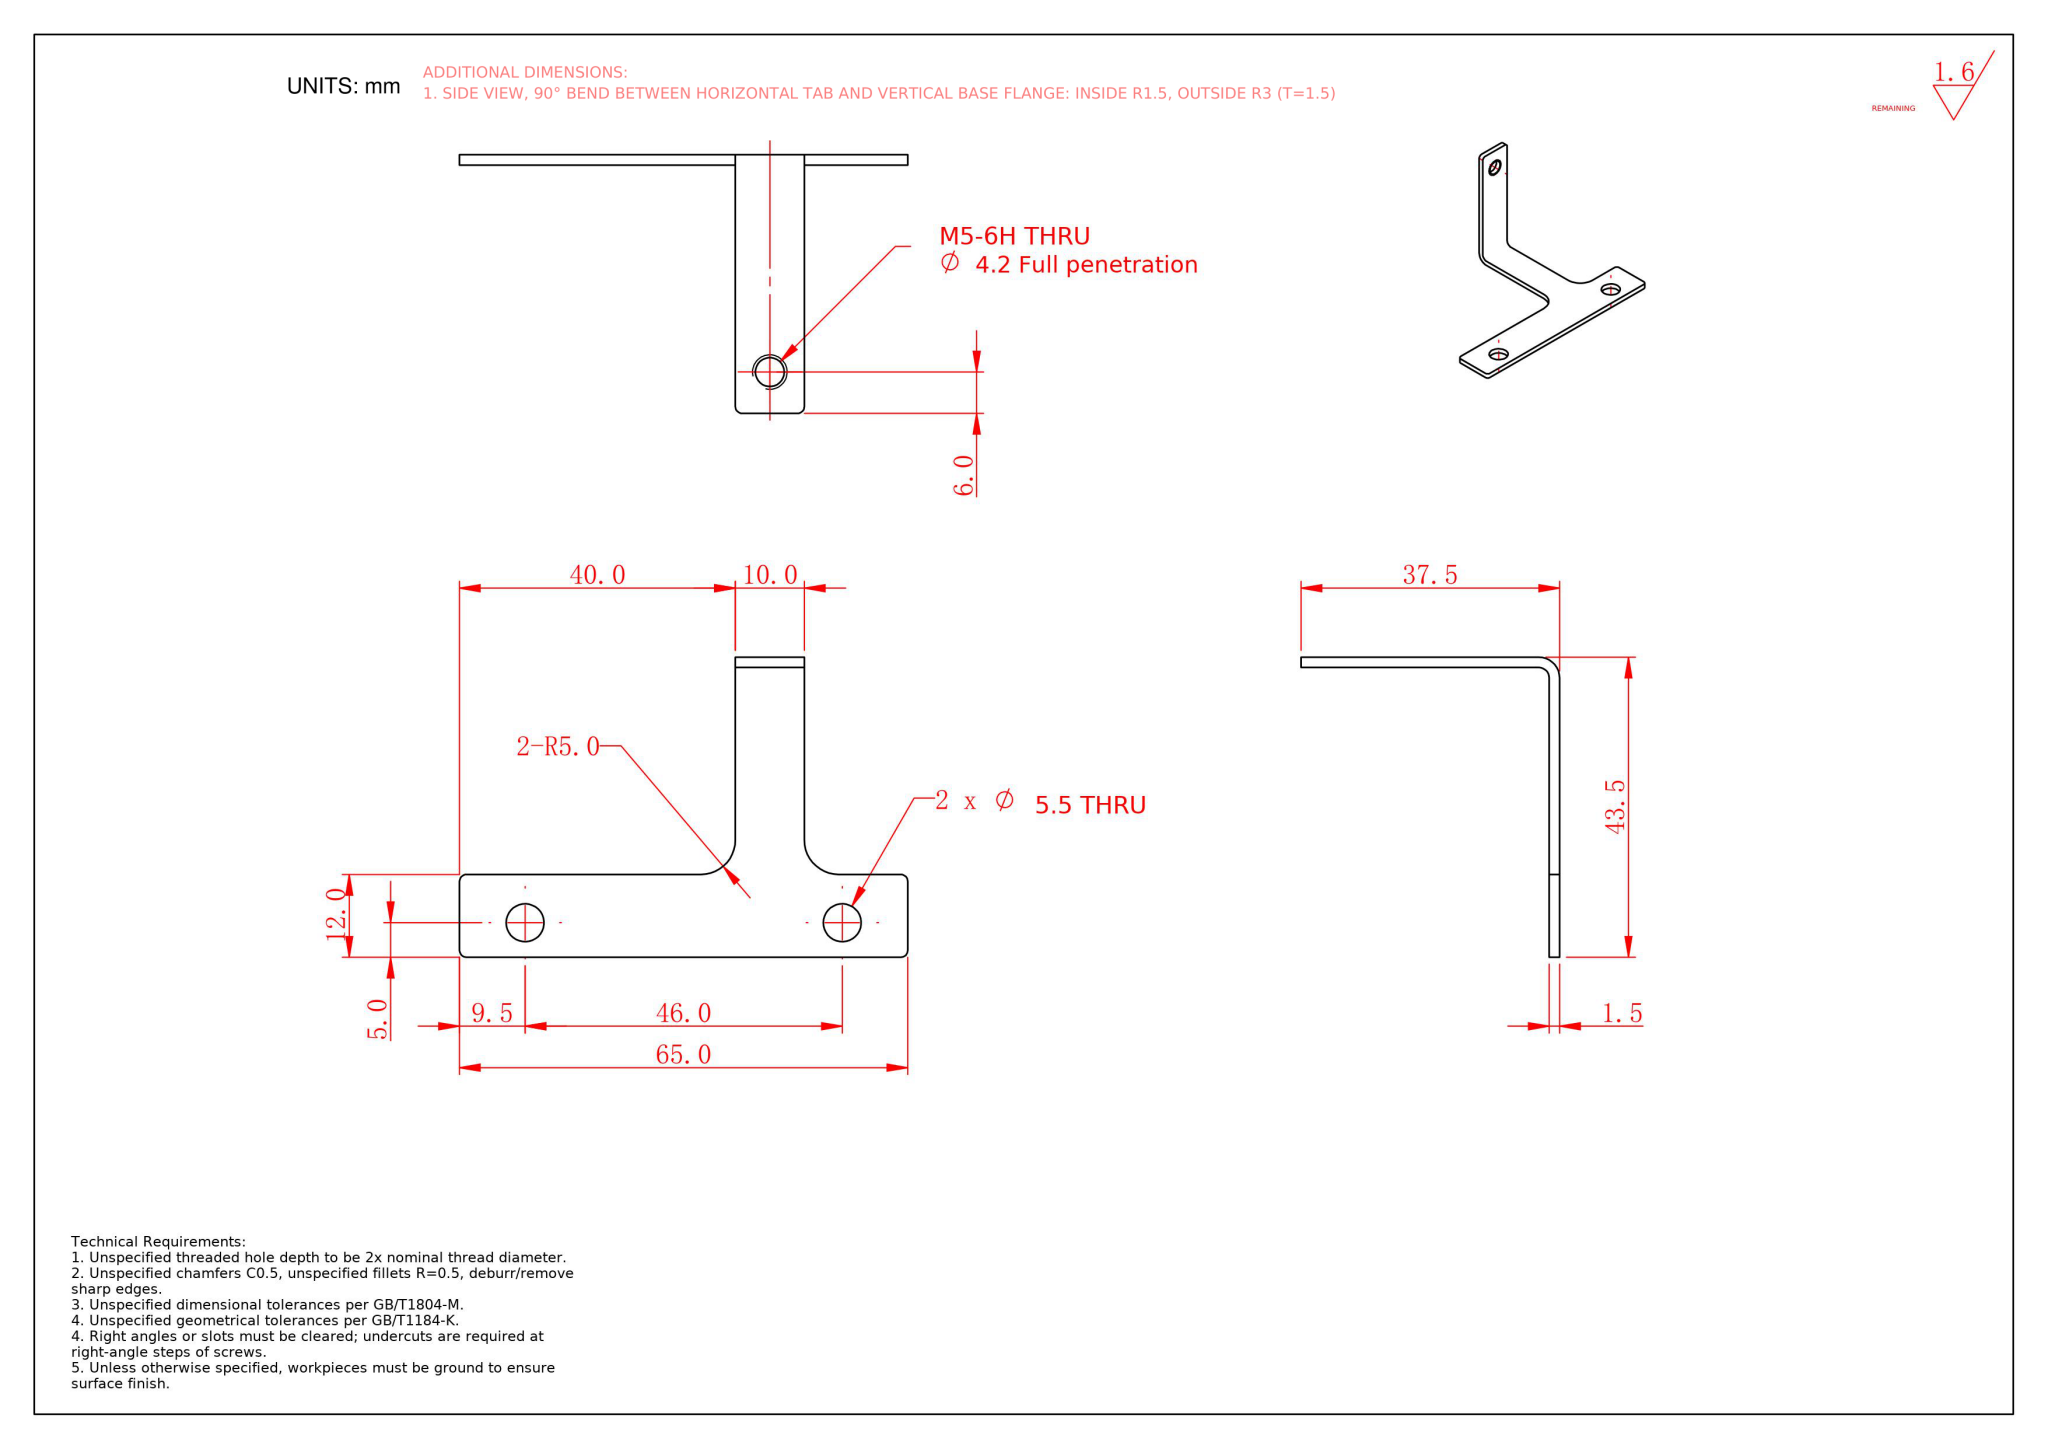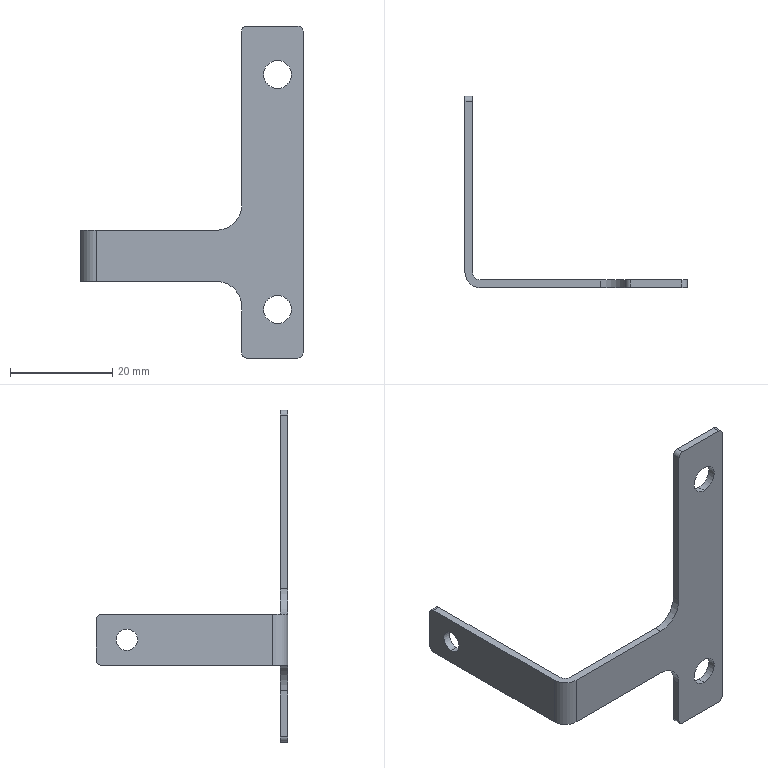Part | NX | mm | 1 solid | 28 faces | box 43.5 x 37.5 x 65 mm | volume 2090 mm3 | cylinder 16 | plane 12 | commonest cylinder face diameters 2 x6 5.5 x4 4.2 x2 10 x2 3 x1 6 x1
STEP:
#1=COLOUR_RGB('',1.,1.,1.);
#2=FILL_AREA_STYLE_COLOUR('',#1);
#3=FILL_AREA_STYLE('',(#2));
#4=SURFACE_STYLE_FILL_AREA(#3);
#5=SURFACE_SIDE_STYLE('',(#4));
#6=SURFACE_STYLE_USAGE(.BOTH.,#5);
#7=PRESENTATION_STYLE_ASSIGNMENT((#6));
#8=CARTESIAN_POINT('',(-27.384,150.278,52.75));
#9=VERTEX_POINT('',#8);
#10=CARTESIAN_POINT('',(-27.384,150.278,58.25));
#11=VERTEX_POINT('',#10);
#12=CARTESIAN_POINT('',(-27.384,150.278,55.5));
#13=DIRECTION('',(0.,1.,0.));
#14=DIRECTION('',(0.,0.,1.));
#15=AXIS2_PLACEMENT_3D('',#12,#13,#14);
#16=CIRCLE('',#15,2.75);
#17=EDGE_CURVE('',#9,#11,#16,.T.);
#18=ORIENTED_EDGE('',*,*,#17,.F.);
#19=CARTESIAN_POINT('',(-27.384,151.778,52.75));
#20=VERTEX_POINT('',#19);
#21=CARTESIAN_POINT('',(-27.384,151.778,52.75));
#22=DIRECTION('',(0.,1.,0.));
#23=VECTOR('',#22,1000.);
#24=LINE('',#21,#23);
#25=EDGE_CURVE('',#9,#20,#24,.T.);
#26=ORIENTED_EDGE('',*,*,#25,.T.);
#27=CARTESIAN_POINT('',(-27.384,151.778,58.25));
#28=VERTEX_POINT('',#27);
#29=CARTESIAN_POINT('',(-27.384,151.778,55.5));
#30=DIRECTION('',(0.,1.,0.));
#31=DIRECTION('',(0.,0.,1.));
#32=AXIS2_PLACEMENT_3D('',#29,#30,#31);
#33=CIRCLE('',#32,2.75);
#34=EDGE_CURVE('',#20,#28,#33,.T.);
#35=ORIENTED_EDGE('',*,*,#34,.T.);
#36=CARTESIAN_POINT('',(-27.384,151.778,58.25));
#37=DIRECTION('',(0.,1.,0.));
#38=VECTOR('',#37,1000.);
#39=LINE('',#36,#38);
#40=EDGE_CURVE('',#11,#28,#39,.T.);
#41=ORIENTED_EDGE('',*,*,#40,.F.);
#42=EDGE_LOOP('',(#18,#26,#35,#41));
#43=FACE_OUTER_BOUND('',#42,.T.);
#44=CARTESIAN_POINT('',(-27.384,151.778,55.5));
#45=DIRECTION('',(0.,1.,0.));
#46=DIRECTION('',(0.,0.,1.));
#47=AXIS2_PLACEMENT_3D('',#44,#45,#46);
#48=CYLINDRICAL_SURFACE('',#47,2.75);
#49=ADVANCED_FACE('',(#43),#48,.F.);
#50=CARTESIAN_POINT('',(-27.384,150.278,6.75));
#51=VERTEX_POINT('',#50);
#52=CARTESIAN_POINT('',(-27.384,150.278,12.25));
#53=VERTEX_POINT('',#52);
#54=CARTESIAN_POINT('',(-27.384,150.278,9.5));
#55=DIRECTION('',(0.,1.,0.));
#56=DIRECTION('',(0.,0.,1.));
#57=AXIS2_PLACEMENT_3D('',#54,#55,#56);
#58=CIRCLE('',#57,2.75);
#59=EDGE_CURVE('',#51,#53,#58,.T.);
#60=ORIENTED_EDGE('',*,*,#59,.F.);
#61=CARTESIAN_POINT('',(-27.384,151.778,6.75));
#62=VERTEX_POINT('',#61);
#63=CARTESIAN_POINT('',(-27.384,151.778,6.75));
#64=DIRECTION('',(0.,1.,0.));
#65=VECTOR('',#64,1000.);
#66=LINE('',#63,#65);
#67=EDGE_CURVE('',#51,#62,#66,.T.);
#68=ORIENTED_EDGE('',*,*,#67,.T.);
#69=CARTESIAN_POINT('',(-27.384,151.778,12.25));
#70=VERTEX_POINT('',#69);
#71=CARTESIAN_POINT('',(-27.384,151.778,9.5));
#72=DIRECTION('',(0.,1.,0.));
#73=DIRECTION('',(0.,0.,1.));
#74=AXIS2_PLACEMENT_3D('',#71,#72,#73);
#75=CIRCLE('',#74,2.75);
#76=EDGE_CURVE('',#62,#70,#75,.T.);
#77=ORIENTED_EDGE('',*,*,#76,.T.);
#78=CARTESIAN_POINT('',(-27.384,151.778,12.25));
#79=DIRECTION('',(0.,1.,0.));
#80=VECTOR('',#79,1000.);
#81=LINE('',#78,#80);
#82=EDGE_CURVE('',#53,#70,#81,.T.);
#83=ORIENTED_EDGE('',*,*,#82,.F.);
#84=EDGE_LOOP('',(#60,#68,#77,#83));
#85=FACE_OUTER_BOUND('',#84,.T.);
#86=CARTESIAN_POINT('',(-27.384,151.778,9.5));
#87=DIRECTION('',(0.,1.,0.));
#88=DIRECTION('',(0.,0.,1.));
#89=AXIS2_PLACEMENT_3D('',#86,#87,#88);
#90=CYLINDRICAL_SURFACE('',#89,2.75);
#91=ADVANCED_FACE('',(#85),#90,.F.);
#92=CARTESIAN_POINT('',(-65.884,181.778,22.1));
#93=VERTEX_POINT('',#92);
#94=CARTESIAN_POINT('',(-65.884,181.778,17.9));
#95=VERTEX_POINT('',#94);
#96=CARTESIAN_POINT('',(-65.884,181.778,20.));
#97=DIRECTION('',(1.,0.,0.));
#98=DIRECTION('',(0.,0.,-1.));
#99=AXIS2_PLACEMENT_3D('',#96,#97,#98);
#100=CIRCLE('',#99,2.1);
#101=EDGE_CURVE('',#93,#95,#100,.T.);
#102=ORIENTED_EDGE('',*,*,#101,.F.);
#103=CARTESIAN_POINT('',(-64.384,181.778,22.1));
#104=VERTEX_POINT('',#103);
#105=CARTESIAN_POINT('',(-64.384,181.778,22.1));
#106=DIRECTION('',(1.,0.,0.));
#107=VECTOR('',#106,1000.);
#108=LINE('',#105,#107);
#109=EDGE_CURVE('',#93,#104,#108,.T.);
#110=ORIENTED_EDGE('',*,*,#109,.T.);
#111=CARTESIAN_POINT('',(-64.384,181.778,17.9));
#112=VERTEX_POINT('',#111);
#113=CARTESIAN_POINT('',(-64.384,181.778,20.));
#114=DIRECTION('',(1.,0.,0.));
#115=DIRECTION('',(0.,0.,-1.));
#116=AXIS2_PLACEMENT_3D('',#113,#114,#115);
#117=CIRCLE('',#116,2.1);
#118=EDGE_CURVE('',#104,#112,#117,.T.);
#119=ORIENTED_EDGE('',*,*,#118,.T.);
#120=CARTESIAN_POINT('',(-64.384,181.778,17.9));
#121=DIRECTION('',(1.,0.,0.));
#122=VECTOR('',#121,1000.);
#123=LINE('',#120,#122);
#124=EDGE_CURVE('',#95,#112,#123,.T.);
#125=ORIENTED_EDGE('',*,*,#124,.F.);
#126=EDGE_LOOP('',(#102,#110,#119,#125));
#127=FACE_OUTER_BOUND('',#126,.T.);
#128=CARTESIAN_POINT('',(-64.384,181.778,20.));
#129=DIRECTION('',(1.,0.,0.));
#130=DIRECTION('',(0.,0.,-1.));
#131=AXIS2_PLACEMENT_3D('',#128,#129,#130);
#132=CYLINDRICAL_SURFACE('',#131,2.1);
#133=ADVANCED_FACE('',(#127),#132,.F.);
#134=CARTESIAN_POINT('',(-33.384,151.778,65.));
#135=VERTEX_POINT('',#134);
#136=CARTESIAN_POINT('',(-23.384,151.778,65.));
#137=VERTEX_POINT('',#136);
#138=CARTESIAN_POINT('',(-64.384,151.778,65.));
#139=DIRECTION('',(1.,0.,0.));
#140=VECTOR('',#139,1000.);
#141=LINE('',#138,#140);
#142=EDGE_CURVE('',#135,#137,#141,.T.);
#143=ORIENTED_EDGE('',*,*,#142,.F.);
#144=CARTESIAN_POINT('',(-33.384,150.278,65.));
#145=VERTEX_POINT('',#144);
#146=CARTESIAN_POINT('',(-33.384,150.278,65.));
#147=DIRECTION('',(0.,-1.,0.));
#148=VECTOR('',#147,1000.);
#149=LINE('',#146,#148);
#150=EDGE_CURVE('',#135,#145,#149,.T.);
#151=ORIENTED_EDGE('',*,*,#150,.T.);
#152=CARTESIAN_POINT('',(-23.384,150.278,65.));
#153=VERTEX_POINT('',#152);
#154=CARTESIAN_POINT('',(-64.384,150.278,65.));
#155=DIRECTION('',(1.,0.,0.));
#156=VECTOR('',#155,1000.);
#157=LINE('',#154,#156);
#158=EDGE_CURVE('',#145,#153,#157,.T.);
#159=ORIENTED_EDGE('',*,*,#158,.T.);
#160=CARTESIAN_POINT('',(-23.384,153.278,65.));
#161=DIRECTION('',(0.,1.,0.));
#162=VECTOR('',#161,1000.);
#163=LINE('',#160,#162);
#164=EDGE_CURVE('',#153,#137,#163,.T.);
#165=ORIENTED_EDGE('',*,*,#164,.T.);
#166=EDGE_LOOP('',(#143,#151,#159,#165));
#167=FACE_OUTER_BOUND('',#166,.T.);
#168=CARTESIAN_POINT('',(-65.884,153.278,65.));
#169=DIRECTION('',(0.,0.,1.));
#170=DIRECTION('',(1.,0.,0.));
#171=AXIS2_PLACEMENT_3D('',#168,#169,#170);
#172=PLANE('',#171);
#173=ADVANCED_FACE('',(#167),#172,.T.);
#174=CARTESIAN_POINT('',(-27.384,150.278,55.5));
#175=DIRECTION('',(0.,1.,0.));
#176=DIRECTION('',(0.,0.,1.));
#177=AXIS2_PLACEMENT_3D('',#174,#175,#176);
#178=CIRCLE('',#177,2.75);
#179=EDGE_CURVE('',#11,#9,#178,.T.);
#180=ORIENTED_EDGE('',*,*,#179,.T.);
#181=ORIENTED_EDGE('',*,*,#17,.T.);
#182=EDGE_LOOP('',(#180,#181));
#183=FACE_BOUND('',#182,.T.);
#184=CARTESIAN_POINT('',(-27.384,150.278,9.5));
#185=DIRECTION('',(0.,1.,0.));
#186=DIRECTION('',(0.,0.,1.));
#187=AXIS2_PLACEMENT_3D('',#184,#185,#186);
#188=CIRCLE('',#187,2.75);
#189=EDGE_CURVE('',#53,#51,#188,.T.);
#190=ORIENTED_EDGE('',*,*,#189,.T.);
#191=ORIENTED_EDGE('',*,*,#59,.T.);
#192=EDGE_LOOP('',(#190,#191));
#193=FACE_BOUND('',#192,.T.);
#194=CARTESIAN_POINT('',(-33.384,150.278,0.));
#195=VERTEX_POINT('',#194);
#196=CARTESIAN_POINT('',(-23.384,150.278,0.));
#197=VERTEX_POINT('',#196);
#198=CARTESIAN_POINT('',(-64.384,150.278,0.));
#199=DIRECTION('',(1.,0.,0.));
#200=VECTOR('',#199,1000.);
#201=LINE('',#198,#200);
#202=EDGE_CURVE('',#195,#197,#201,.T.);
#203=ORIENTED_EDGE('',*,*,#202,.T.);
#204=CARTESIAN_POINT('',(-22.384,150.278,1.));
#205=VERTEX_POINT('',#204);
#206=CARTESIAN_POINT('',(-23.384,150.278,1.));
#207=DIRECTION('',(0.,-1.,0.));
#208=DIRECTION('',(0.,0.,1.));
#209=AXIS2_PLACEMENT_3D('',#206,#207,#208);
#210=CIRCLE('',#209,1.);
#211=EDGE_CURVE('',#197,#205,#210,.T.);
#212=ORIENTED_EDGE('',*,*,#211,.T.);
#213=CARTESIAN_POINT('',(-22.384,150.278,64.));
#214=VERTEX_POINT('',#213);
#215=CARTESIAN_POINT('',(-22.384,150.278,65.));
#216=DIRECTION('',(0.,0.,-1.));
#217=VECTOR('',#216,1000.);
#218=LINE('',#215,#217);
#219=EDGE_CURVE('',#214,#205,#218,.T.);
#220=ORIENTED_EDGE('',*,*,#219,.F.);
#221=CARTESIAN_POINT('',(-23.384,150.278,64.));
#222=DIRECTION('',(0.,-1.,0.));
#223=DIRECTION('',(0.,0.,1.));
#224=AXIS2_PLACEMENT_3D('',#221,#222,#223);
#225=CIRCLE('',#224,1.);
#226=EDGE_CURVE('',#214,#153,#225,.T.);
#227=ORIENTED_EDGE('',*,*,#226,.T.);
#228=ORIENTED_EDGE('',*,*,#158,.F.);
#229=CARTESIAN_POINT('',(-34.384,150.278,64.));
#230=VERTEX_POINT('',#229);
#231=CARTESIAN_POINT('',(-33.384,150.278,64.));
#232=DIRECTION('',(0.,-1.,0.));
#233=DIRECTION('',(0.,0.,1.));
#234=AXIS2_PLACEMENT_3D('',#231,#232,#233);
#235=CIRCLE('',#234,1.);
#236=EDGE_CURVE('',#145,#230,#235,.T.);
#237=ORIENTED_EDGE('',*,*,#236,.T.);
#238=CARTESIAN_POINT('',(-34.384,150.278,30.));
#239=VERTEX_POINT('',#238);
#240=CARTESIAN_POINT('',(-34.384,150.278,79.419));
#241=DIRECTION('',(-0.,0.,-1.));
#242=VECTOR('',#241,1000.);
#243=LINE('',#240,#242);
#244=EDGE_CURVE('',#230,#239,#243,.T.);
#245=ORIENTED_EDGE('',*,*,#244,.T.);
#246=CARTESIAN_POINT('',(-39.384,150.278,25.));
#247=VERTEX_POINT('',#246);
#248=CARTESIAN_POINT('',(-39.384,150.278,30.));
#249=DIRECTION('',(0.,1.,0.));
#250=DIRECTION('',(0.,0.,1.));
#251=AXIS2_PLACEMENT_3D('',#248,#249,#250);
#252=CIRCLE('',#251,5.);
#253=EDGE_CURVE('',#239,#247,#252,.T.);
#254=ORIENTED_EDGE('',*,*,#253,.T.);
#255=CARTESIAN_POINT('',(-62.884,150.278,25.));
#256=VERTEX_POINT('',#255);
#257=CARTESIAN_POINT('',(-74.236,150.278,25.));
#258=DIRECTION('',(-1.,0.,0.));
#259=VECTOR('',#258,1000.);
#260=LINE('',#257,#259);
#261=EDGE_CURVE('',#247,#256,#260,.T.);
#262=ORIENTED_EDGE('',*,*,#261,.T.);
#263=CARTESIAN_POINT('',(-62.884,150.278,15.));
#264=VERTEX_POINT('',#263);
#265=CARTESIAN_POINT('',(-62.884,150.278,65.));
#266=DIRECTION('',(0.,0.,-1.));
#267=VECTOR('',#266,1000.);
#268=LINE('',#265,#267);
#269=EDGE_CURVE('',#256,#264,#268,.T.);
#270=ORIENTED_EDGE('',*,*,#269,.T.);
#271=CARTESIAN_POINT('',(-39.384,150.278,15.));
#272=VERTEX_POINT('',#271);
#273=CARTESIAN_POINT('',(-74.236,150.278,15.));
#274=DIRECTION('',(1.,0.,0.));
#275=VECTOR('',#274,1000.);
#276=LINE('',#273,#275);
#277=EDGE_CURVE('',#264,#272,#276,.T.);
#278=ORIENTED_EDGE('',*,*,#277,.T.);
#279=CARTESIAN_POINT('',(-34.384,150.278,10.));
#280=VERTEX_POINT('',#279);
#281=CARTESIAN_POINT('',(-39.384,150.278,10.));
#282=DIRECTION('',(0.,1.,0.));
#283=DIRECTION('',(0.,0.,1.));
#284=AXIS2_PLACEMENT_3D('',#281,#282,#283);
#285=CIRCLE('',#284,5.);
#286=EDGE_CURVE('',#272,#280,#285,.T.);
#287=ORIENTED_EDGE('',*,*,#286,.T.);
#288=CARTESIAN_POINT('',(-34.384,150.278,1.));
#289=VERTEX_POINT('',#288);
#290=CARTESIAN_POINT('',(-34.384,150.278,-20.192));
#291=DIRECTION('',(-0.,0.,-1.));
#292=VECTOR('',#291,1000.);
#293=LINE('',#290,#292);
#294=EDGE_CURVE('',#280,#289,#293,.T.);
#295=ORIENTED_EDGE('',*,*,#294,.T.);
#296=CARTESIAN_POINT('',(-33.384,150.278,1.));
#297=DIRECTION('',(0.,-1.,0.));
#298=DIRECTION('',(0.,0.,1.));
#299=AXIS2_PLACEMENT_3D('',#296,#297,#298);
#300=CIRCLE('',#299,1.);
#301=EDGE_CURVE('',#289,#195,#300,.T.);
#302=ORIENTED_EDGE('',*,*,#301,.T.);
#303=EDGE_LOOP('',(#203,#212,#220,#227,#228,#237,#245,#254,#262,#270,#278,#287,#295,#302));
#304=FACE_OUTER_BOUND('',#303,.T.);
#305=CARTESIAN_POINT('',(-64.384,150.278,65.));
#306=DIRECTION('',(0.,1.,0.));
#307=DIRECTION('',(0.,0.,1.));
#308=AXIS2_PLACEMENT_3D('',#305,#306,#307);
#309=PLANE('',#308);
#310=ADVANCED_FACE('',(#183,#193,#304),#309,.F.);
#311=ORIENTED_EDGE('',*,*,#219,.T.);
#312=CARTESIAN_POINT('',(-22.384,151.778,1.));
#313=VERTEX_POINT('',#312);
#314=CARTESIAN_POINT('',(-22.384,151.778,1.));
#315=DIRECTION('',(0.,1.,0.));
#316=VECTOR('',#315,1000.);
#317=LINE('',#314,#316);
#318=EDGE_CURVE('',#205,#313,#317,.T.);
#319=ORIENTED_EDGE('',*,*,#318,.T.);
#320=CARTESIAN_POINT('',(-22.384,151.778,64.));
#321=VERTEX_POINT('',#320);
#322=CARTESIAN_POINT('',(-22.384,151.778,65.));
#323=DIRECTION('',(0.,0.,-1.));
#324=VECTOR('',#323,1000.);
#325=LINE('',#322,#324);
#326=EDGE_CURVE('',#321,#313,#325,.T.);
#327=ORIENTED_EDGE('',*,*,#326,.F.);
#328=CARTESIAN_POINT('',(-22.384,151.778,64.));
#329=DIRECTION('',(0.,-1.,0.));
#330=VECTOR('',#329,1000.);
#331=LINE('',#328,#330);
#332=EDGE_CURVE('',#321,#214,#331,.T.);
#333=ORIENTED_EDGE('',*,*,#332,.T.);
#334=EDGE_LOOP('',(#311,#319,#327,#333));
#335=FACE_OUTER_BOUND('',#334,.T.);
#336=CARTESIAN_POINT('',(-22.384,151.778,65.));
#337=DIRECTION('',(1.,0.,0.));
#338=DIRECTION('',(0.,0.,-1.));
#339=AXIS2_PLACEMENT_3D('',#336,#337,#338);
#340=PLANE('',#339);
#341=ADVANCED_FACE('',(#335),#340,.T.);
#342=CARTESIAN_POINT('',(-27.384,151.778,55.5));
#343=DIRECTION('',(0.,1.,0.));
#344=DIRECTION('',(0.,0.,1.));
#345=AXIS2_PLACEMENT_3D('',#342,#343,#344);
#346=CIRCLE('',#345,2.75);
#347=EDGE_CURVE('',#28,#20,#346,.T.);
#348=ORIENTED_EDGE('',*,*,#347,.F.);
#349=ORIENTED_EDGE('',*,*,#34,.F.);
#350=EDGE_LOOP('',(#348,#349));
#351=FACE_BOUND('',#350,.T.);
#352=CARTESIAN_POINT('',(-27.384,151.778,9.5));
#353=DIRECTION('',(0.,1.,0.));
#354=DIRECTION('',(0.,0.,1.));
#355=AXIS2_PLACEMENT_3D('',#352,#353,#354);
#356=CIRCLE('',#355,2.75);
#357=EDGE_CURVE('',#70,#62,#356,.T.);
#358=ORIENTED_EDGE('',*,*,#357,.F.);
#359=ORIENTED_EDGE('',*,*,#76,.F.);
#360=EDGE_LOOP('',(#358,#359));
#361=FACE_BOUND('',#360,.T.);
#362=ORIENTED_EDGE('',*,*,#326,.T.);
#363=CARTESIAN_POINT('',(-23.384,151.778,0.));
#364=VERTEX_POINT('',#363);
#365=CARTESIAN_POINT('',(-23.384,151.778,1.));
#366=DIRECTION('',(0.,1.,0.));
#367=DIRECTION('',(0.,0.,1.));
#368=AXIS2_PLACEMENT_3D('',#365,#366,#367);
#369=CIRCLE('',#368,1.);
#370=EDGE_CURVE('',#313,#364,#369,.T.);
#371=ORIENTED_EDGE('',*,*,#370,.T.);
#372=CARTESIAN_POINT('',(-33.384,151.778,0.));
#373=VERTEX_POINT('',#372);
#374=CARTESIAN_POINT('',(-64.384,151.778,0.));
#375=DIRECTION('',(1.,0.,0.));
#376=VECTOR('',#375,1000.);
#377=LINE('',#374,#376);
#378=EDGE_CURVE('',#373,#364,#377,.T.);
#379=ORIENTED_EDGE('',*,*,#378,.F.);
#380=CARTESIAN_POINT('',(-34.384,151.778,1.));
#381=VERTEX_POINT('',#380);
#382=CARTESIAN_POINT('',(-33.384,151.778,1.));
#383=DIRECTION('',(0.,1.,0.));
#384=DIRECTION('',(0.,0.,1.));
#385=AXIS2_PLACEMENT_3D('',#382,#383,#384);
#386=CIRCLE('',#385,1.);
#387=EDGE_CURVE('',#373,#381,#386,.T.);
#388=ORIENTED_EDGE('',*,*,#387,.T.);
#389=CARTESIAN_POINT('',(-34.384,151.778,10.));
#390=VERTEX_POINT('',#389);
#391=CARTESIAN_POINT('',(-34.384,151.778,65.));
#392=DIRECTION('',(-0.,0.,-1.));
#393=VECTOR('',#392,1000.);
#394=LINE('',#391,#393);
#395=EDGE_CURVE('',#390,#381,#394,.T.);
#396=ORIENTED_EDGE('',*,*,#395,.F.);
#397=CARTESIAN_POINT('',(-39.384,151.778,15.));
#398=VERTEX_POINT('',#397);
#399=CARTESIAN_POINT('',(-39.384,151.778,10.));
#400=DIRECTION('',(0.,-1.,0.));
#401=DIRECTION('',(-0.,0.,1.));
#402=AXIS2_PLACEMENT_3D('',#399,#400,#401);
#403=CIRCLE('',#402,5.);
#404=EDGE_CURVE('',#390,#398,#403,.T.);
#405=ORIENTED_EDGE('',*,*,#404,.T.);
#406=CARTESIAN_POINT('',(-62.884,151.778,15.));
#407=VERTEX_POINT('',#406);
#408=CARTESIAN_POINT('',(-64.384,151.778,15.));
#409=DIRECTION('',(1.,0.,0.));
#410=VECTOR('',#409,1000.);
#411=LINE('',#408,#410);
#412=EDGE_CURVE('',#407,#398,#411,.T.);
#413=ORIENTED_EDGE('',*,*,#412,.F.);
#414=CARTESIAN_POINT('',(-62.884,151.778,25.));
#415=VERTEX_POINT('',#414);
#416=CARTESIAN_POINT('',(-62.884,151.778,65.));
#417=DIRECTION('',(0.,0.,-1.));
#418=VECTOR('',#417,1000.);
#419=LINE('',#416,#418);
#420=EDGE_CURVE('',#415,#407,#419,.T.);
#421=ORIENTED_EDGE('',*,*,#420,.F.);
#422=CARTESIAN_POINT('',(-39.384,151.778,25.));
#423=VERTEX_POINT('',#422);
#424=CARTESIAN_POINT('',(-64.384,151.778,25.));
#425=DIRECTION('',(-1.,0.,0.));
#426=VECTOR('',#425,1000.);
#427=LINE('',#424,#426);
#428=EDGE_CURVE('',#423,#415,#427,.T.);
#429=ORIENTED_EDGE('',*,*,#428,.F.);
#430=CARTESIAN_POINT('',(-34.384,151.778,30.));
#431=VERTEX_POINT('',#430);
#432=CARTESIAN_POINT('',(-39.384,151.778,30.));
#433=DIRECTION('',(0.,-1.,0.));
#434=DIRECTION('',(0.,0.,1.));
#435=AXIS2_PLACEMENT_3D('',#432,#433,#434);
#436=CIRCLE('',#435,5.);
#437=EDGE_CURVE('',#423,#431,#436,.T.);
#438=ORIENTED_EDGE('',*,*,#437,.T.);
#439=CARTESIAN_POINT('',(-34.384,151.778,64.));
#440=VERTEX_POINT('',#439);
#441=CARTESIAN_POINT('',(-34.384,151.778,65.));
#442=DIRECTION('',(-0.,0.,-1.));
#443=VECTOR('',#442,1000.);
#444=LINE('',#441,#443);
#445=EDGE_CURVE('',#440,#431,#444,.T.);
#446=ORIENTED_EDGE('',*,*,#445,.F.);
#447=CARTESIAN_POINT('',(-33.384,151.778,64.));
#448=DIRECTION('',(0.,1.,0.));
#449=DIRECTION('',(0.,0.,1.));
#450=AXIS2_PLACEMENT_3D('',#447,#448,#449);
#451=CIRCLE('',#450,1.);
#452=EDGE_CURVE('',#440,#135,#451,.T.);
#453=ORIENTED_EDGE('',*,*,#452,.T.);
#454=ORIENTED_EDGE('',*,*,#142,.T.);
#455=CARTESIAN_POINT('',(-23.384,151.778,64.));
#456=DIRECTION('',(0.,1.,0.));
#457=DIRECTION('',(0.,0.,1.));
#458=AXIS2_PLACEMENT_3D('',#455,#456,#457);
#459=CIRCLE('',#458,1.);
#460=EDGE_CURVE('',#137,#321,#459,.T.);
#461=ORIENTED_EDGE('',*,*,#460,.T.);
#462=EDGE_LOOP('',(#362,#371,#379,#388,#396,#405,#413,#421,#429,#438,#446,#453,#454,#461));
#463=FACE_OUTER_BOUND('',#462,.T.);
#464=CARTESIAN_POINT('',(-64.384,151.778,65.));
#465=DIRECTION('',(0.,1.,0.));
#466=DIRECTION('',(0.,0.,1.));
#467=AXIS2_PLACEMENT_3D('',#464,#465,#466);
#468=PLANE('',#467);
#469=ADVANCED_FACE('',(#351,#361,#463),#468,.T.);
#470=CARTESIAN_POINT('',(-64.384,153.278,25.));
#471=VERTEX_POINT('',#470);
#472=CARTESIAN_POINT('',(-62.884,153.278,25.));
#473=DIRECTION('',(0.,0.,-1.));
#474=DIRECTION('',(-1.,0.,0.));
#475=AXIS2_PLACEMENT_3D('',#472,#473,#474);
#476=CIRCLE('',#475,1.5);
#477=EDGE_CURVE('',#415,#471,#476,.T.);
#478=ORIENTED_EDGE('',*,*,#477,.F.);
#479=ORIENTED_EDGE('',*,*,#420,.T.);
#480=CARTESIAN_POINT('',(-64.384,153.278,15.));
#481=VERTEX_POINT('',#480);
#482=CARTESIAN_POINT('',(-62.884,153.278,15.));
#483=DIRECTION('',(0.,0.,1.));
#484=DIRECTION('',(1.,0.,0.));
#485=AXIS2_PLACEMENT_3D('',#482,#483,#484);
#486=CIRCLE('',#485,1.5);
#487=EDGE_CURVE('',#481,#407,#486,.T.);
#488=ORIENTED_EDGE('',*,*,#487,.F.);
#489=CARTESIAN_POINT('',(-64.384,153.278,65.));
#490=DIRECTION('',(0.,0.,-1.));
#491=VECTOR('',#490,1000.);
#492=LINE('',#489,#491);
#493=EDGE_CURVE('',#471,#481,#492,.T.);
#494=ORIENTED_EDGE('',*,*,#493,.F.);
#495=EDGE_LOOP('',(#478,#479,#488,#494));
#496=FACE_OUTER_BOUND('',#495,.T.);
#497=CARTESIAN_POINT('',(-62.884,153.278,65.));
#498=DIRECTION('',(0.,0.,-1.));
#499=DIRECTION('',(-1.,0.,0.));
#500=AXIS2_PLACEMENT_3D('',#497,#498,#499);
#501=CYLINDRICAL_SURFACE('',#500,1.5);
#502=ADVANCED_FACE('',(#496),#501,.F.);
#503=CARTESIAN_POINT('',(-64.384,181.778,20.));
#504=DIRECTION('',(1.,0.,0.));
#505=DIRECTION('',(0.,0.,-1.));
#506=AXIS2_PLACEMENT_3D('',#503,#504,#505);
#507=CIRCLE('',#506,2.1);
#508=EDGE_CURVE('',#112,#104,#507,.T.);
#509=ORIENTED_EDGE('',*,*,#508,.F.);
#510=ORIENTED_EDGE('',*,*,#118,.F.);
#511=EDGE_LOOP('',(#509,#510));
#512=FACE_BOUND('',#511,.T.);
#513=CARTESIAN_POINT('',(-64.384,186.778,15.));
#514=VERTEX_POINT('',#513);
#515=CARTESIAN_POINT('',(-64.384,187.778,15.));
#516=DIRECTION('',(0.,-1.,0.));
#517=VECTOR('',#516,1000.);
#518=LINE('',#515,#517);
#519=EDGE_CURVE('',#514,#481,#518,.T.);
#520=ORIENTED_EDGE('',*,*,#519,.F.);
#521=CARTESIAN_POINT('',(-64.384,187.778,16.));
#522=VERTEX_POINT('',#521);
#523=CARTESIAN_POINT('',(-64.384,186.778,16.));
#524=DIRECTION('',(1.,0.,0.));
#525=DIRECTION('',(0.,1.,0.));
#526=AXIS2_PLACEMENT_3D('',#523,#524,#525);
#527=CIRCLE('',#526,1.);
#528=EDGE_CURVE('',#514,#522,#527,.T.);
#529=ORIENTED_EDGE('',*,*,#528,.T.);
#530=CARTESIAN_POINT('',(-64.384,187.778,24.));
#531=VERTEX_POINT('',#530);
#532=CARTESIAN_POINT('',(-64.384,187.778,65.));
#533=DIRECTION('',(0.,0.,-1.));
#534=VECTOR('',#533,1000.);
#535=LINE('',#532,#534);
#536=EDGE_CURVE('',#531,#522,#535,.T.);
#537=ORIENTED_EDGE('',*,*,#536,.F.);
#538=CARTESIAN_POINT('',(-64.384,186.778,25.));
#539=VERTEX_POINT('',#538);
#540=CARTESIAN_POINT('',(-64.384,186.778,24.));
#541=DIRECTION('',(1.,0.,0.));
#542=DIRECTION('',(0.,1.,0.));
#543=AXIS2_PLACEMENT_3D('',#540,#541,#542);
#544=CIRCLE('',#543,1.);
#545=EDGE_CURVE('',#531,#539,#544,.T.);
#546=ORIENTED_EDGE('',*,*,#545,.T.);
#547=CARTESIAN_POINT('',(-64.384,187.778,25.));
#548=DIRECTION('',(-0.,1.,0.));
#549=VECTOR('',#548,1000.);
#550=LINE('',#547,#549);
#551=EDGE_CURVE('',#471,#539,#550,.T.);
#552=ORIENTED_EDGE('',*,*,#551,.F.);
#553=ORIENTED_EDGE('',*,*,#493,.T.);
#554=EDGE_LOOP('',(#520,#529,#537,#546,#552,#553));
#555=FACE_OUTER_BOUND('',#554,.T.);
#556=CARTESIAN_POINT('',(-64.384,187.778,65.));
#557=DIRECTION('',(1.,0.,0.));
#558=DIRECTION('',(-0.,1.,0.));
#559=AXIS2_PLACEMENT_3D('',#556,#557,#558);
#560=PLANE('',#559);
#561=ADVANCED_FACE('',(#512,#555),#560,.T.);
#562=ORIENTED_EDGE('',*,*,#536,.T.);
#563=CARTESIAN_POINT('',(-65.884,187.778,16.));
#564=VERTEX_POINT('',#563);
#565=CARTESIAN_POINT('',(-65.884,187.778,16.));
#566=DIRECTION('',(-1.,0.,0.));
#567=VECTOR('',#566,1000.);
#568=LINE('',#565,#567);
#569=EDGE_CURVE('',#522,#564,#568,.T.);
#570=ORIENTED_EDGE('',*,*,#569,.T.);
#571=CARTESIAN_POINT('',(-65.884,187.778,24.));
#572=VERTEX_POINT('',#571);
#573=CARTESIAN_POINT('',(-65.884,187.778,65.));
#574=DIRECTION('',(0.,0.,-1.));
#575=VECTOR('',#574,1000.);
#576=LINE('',#573,#575);
#577=EDGE_CURVE('',#572,#564,#576,.T.);
#578=ORIENTED_EDGE('',*,*,#577,.F.);
#579=CARTESIAN_POINT('',(-64.384,187.778,24.));
#580=DIRECTION('',(1.,0.,0.));
#581=VECTOR('',#580,1000.);
#582=LINE('',#579,#581);
#583=EDGE_CURVE('',#572,#531,#582,.T.);
#584=ORIENTED_EDGE('',*,*,#583,.T.);
#585=EDGE_LOOP('',(#562,#570,#578,#584));
#586=FACE_OUTER_BOUND('',#585,.T.);
#587=CARTESIAN_POINT('',(-65.884,187.778,65.));
#588=DIRECTION('',(0.,1.,0.));
#589=DIRECTION('',(0.,0.,1.));
#590=AXIS2_PLACEMENT_3D('',#587,#588,#589);
#591=PLANE('',#590);
#592=ADVANCED_FACE('',(#586),#591,.T.);
#593=CARTESIAN_POINT('',(-65.884,181.778,20.));
#594=DIRECTION('',(1.,0.,0.));
#595=DIRECTION('',(0.,0.,-1.));
#596=AXIS2_PLACEMENT_3D('',#593,#594,#595);
#597=CIRCLE('',#596,2.1);
#598=EDGE_CURVE('',#95,#93,#597,.T.);
#599=ORIENTED_EDGE('',*,*,#598,.T.);
#600=ORIENTED_EDGE('',*,*,#101,.T.);
#601=EDGE_LOOP('',(#599,#600));
#602=FACE_BOUND('',#601,.T.);
#603=ORIENTED_EDGE('',*,*,#577,.T.);
#604=CARTESIAN_POINT('',(-65.884,186.778,15.));
#605=VERTEX_POINT('',#604);
#606=CARTESIAN_POINT('',(-65.884,186.778,16.));
#607=DIRECTION('',(-1.,-0.,0.));
#608=DIRECTION('',(0.,1.,0.));
#609=AXIS2_PLACEMENT_3D('',#606,#607,#608);
#610=CIRCLE('',#609,1.);
#611=EDGE_CURVE('',#564,#605,#610,.T.);
#612=ORIENTED_EDGE('',*,*,#611,.T.);
#613=CARTESIAN_POINT('',(-65.884,153.278,15.));
#614=VERTEX_POINT('',#613);
#615=CARTESIAN_POINT('',(-65.884,187.778,15.));
#616=DIRECTION('',(0.,-1.,0.));
#617=VECTOR('',#616,1000.);
#618=LINE('',#615,#617);
#619=EDGE_CURVE('',#605,#614,#618,.T.);
#620=ORIENTED_EDGE('',*,*,#619,.T.);
#621=CARTESIAN_POINT('',(-65.884,153.278,25.));
#622=VERTEX_POINT('',#621);
#623=CARTESIAN_POINT('',(-65.884,153.278,65.));
#624=DIRECTION('',(0.,0.,-1.));
#625=VECTOR('',#624,1000.);
#626=LINE('',#623,#625);
#627=EDGE_CURVE('',#622,#614,#626,.T.);
#628=ORIENTED_EDGE('',*,*,#627,.F.);
#629=CARTESIAN_POINT('',(-65.884,186.778,25.));
#630=VERTEX_POINT('',#629);
#631=CARTESIAN_POINT('',(-65.884,187.778,25.));
#632=DIRECTION('',(-0.,1.,0.));
#633=VECTOR('',#632,1000.);
#634=LINE('',#631,#633);
#635=EDGE_CURVE('',#622,#630,#634,.T.);
#636=ORIENTED_EDGE('',*,*,#635,.T.);
#637=CARTESIAN_POINT('',(-65.884,186.778,24.));
#638=DIRECTION('',(-1.,-0.,0.));
#639=DIRECTION('',(0.,1.,0.));
#640=AXIS2_PLACEMENT_3D('',#637,#638,#639);
#641=CIRCLE('',#640,1.);
#642=EDGE_CURVE('',#630,#572,#641,.T.);
#643=ORIENTED_EDGE('',*,*,#642,.T.);
#644=EDGE_LOOP('',(#603,#612,#620,#628,#636,#643));
#645=FACE_OUTER_BOUND('',#644,.T.);
#646=CARTESIAN_POINT('',(-65.884,187.778,65.));
#647=DIRECTION('',(1.,0.,0.));
#648=DIRECTION('',(-0.,1.,0.));
#649=AXIS2_PLACEMENT_3D('',#646,#647,#648);
#650=PLANE('',#649);
#651=ADVANCED_FACE('',(#602,#645),#650,.F.);
#652=ORIENTED_EDGE('',*,*,#269,.F.);
#653=CARTESIAN_POINT('',(-62.884,153.278,25.));
#654=DIRECTION('',(0.,0.,-1.));
#655=DIRECTION('',(-1.,0.,0.));
#656=AXIS2_PLACEMENT_3D('',#653,#654,#655);
#657=CIRCLE('',#656,3.);
#658=EDGE_CURVE('',#256,#622,#657,.T.);
#659=ORIENTED_EDGE('',*,*,#658,.T.);
#660=ORIENTED_EDGE('',*,*,#627,.T.);
#661=CARTESIAN_POINT('',(-62.884,153.278,15.));
#662=DIRECTION('',(0.,0.,1.));
#663=DIRECTION('',(1.,0.,0.));
#664=AXIS2_PLACEMENT_3D('',#661,#662,#663);
#665=CIRCLE('',#664,3.);
#666=EDGE_CURVE('',#614,#264,#665,.T.);
#667=ORIENTED_EDGE('',*,*,#666,.T.);
#668=EDGE_LOOP('',(#652,#659,#660,#667));
#669=FACE_OUTER_BOUND('',#668,.T.);
#670=CARTESIAN_POINT('',(-62.884,153.278,65.));
#671=DIRECTION('',(0.,0.,-1.));
#672=DIRECTION('',(-1.,0.,0.));
#673=AXIS2_PLACEMENT_3D('',#670,#671,#672);
#674=CYLINDRICAL_SURFACE('',#673,3.);
#675=ADVANCED_FACE('',(#669),#674,.T.);
#676=ORIENTED_EDGE('',*,*,#378,.T.);
#677=CARTESIAN_POINT('',(-23.384,153.278,0.));
#678=DIRECTION('',(0.,-1.,0.));
#679=VECTOR('',#678,1000.);
#680=LINE('',#677,#679);
#681=EDGE_CURVE('',#364,#197,#680,.T.);
#682=ORIENTED_EDGE('',*,*,#681,.T.);
#683=ORIENTED_EDGE('',*,*,#202,.F.);
#684=CARTESIAN_POINT('',(-33.384,151.778,0.));
#685=DIRECTION('',(0.,1.,0.));
#686=VECTOR('',#685,1000.);
#687=LINE('',#684,#686);
#688=EDGE_CURVE('',#195,#373,#687,.T.);
#689=ORIENTED_EDGE('',*,*,#688,.T.);
#690=EDGE_LOOP('',(#676,#682,#683,#689));
#691=FACE_OUTER_BOUND('',#690,.T.);
#692=CARTESIAN_POINT('',(-62.884,153.278,0.));
#693=DIRECTION('',(0.,0.,-1.));
#694=DIRECTION('',(-1.,0.,0.));
#695=AXIS2_PLACEMENT_3D('',#692,#693,#694);
#696=PLANE('',#695);
#697=ADVANCED_FACE('',(#691),#696,.T.);
#698=ORIENTED_EDGE('',*,*,#412,.T.);
#699=CARTESIAN_POINT('',(-39.384,150.278,15.));
#700=DIRECTION('',(0.,-1.,0.));
#701=VECTOR('',#700,1000.);
#702=LINE('',#699,#701);
#703=EDGE_CURVE('',#398,#272,#702,.T.);
#704=ORIENTED_EDGE('',*,*,#703,.T.);
#705=ORIENTED_EDGE('',*,*,#277,.F.);
#706=ORIENTED_EDGE('',*,*,#666,.F.);
#707=ORIENTED_EDGE('',*,*,#619,.F.);
#708=CARTESIAN_POINT('',(-64.384,186.778,15.));
#709=DIRECTION('',(1.,0.,0.));
#710=VECTOR('',#709,1000.);
#711=LINE('',#708,#710);
#712=EDGE_CURVE('',#605,#514,#711,.T.);
#713=ORIENTED_EDGE('',*,*,#712,.T.);
#714=ORIENTED_EDGE('',*,*,#519,.T.);
#715=ORIENTED_EDGE('',*,*,#487,.T.);
#716=EDGE_LOOP('',(#698,#704,#705,#706,#707,#713,#714,#715));
#717=FACE_OUTER_BOUND('',#716,.T.);
#718=CARTESIAN_POINT('',(-74.236,150.278,15.));
#719=DIRECTION('',(0.,0.,1.));
#720=DIRECTION('',(1.,0.,0.));
#721=AXIS2_PLACEMENT_3D('',#718,#719,#720);
#722=PLANE('',#721);
#723=ADVANCED_FACE('',(#717),#722,.F.);
#724=ORIENTED_EDGE('',*,*,#294,.F.);
#725=CARTESIAN_POINT('',(-34.384,151.778,10.));
#726=DIRECTION('',(0.,1.,0.));
#727=VECTOR('',#726,1000.);
#728=LINE('',#725,#727);
#729=EDGE_CURVE('',#280,#390,#728,.T.);
#730=ORIENTED_EDGE('',*,*,#729,.T.);
#731=ORIENTED_EDGE('',*,*,#395,.T.);
#732=CARTESIAN_POINT('',(-34.384,150.278,1.));
#733=DIRECTION('',(0.,-1.,0.));
#734=VECTOR('',#733,1000.);
#735=LINE('',#732,#734);
#736=EDGE_CURVE('',#381,#289,#735,.T.);
#737=ORIENTED_EDGE('',*,*,#736,.T.);
#738=EDGE_LOOP('',(#724,#730,#731,#737));
#739=FACE_OUTER_BOUND('',#738,.T.);
#740=CARTESIAN_POINT('',(-34.384,150.278,-20.192));
#741=DIRECTION('',(1.,0.,-0.));
#742=DIRECTION('',(-0.,0.,-1.));
#743=AXIS2_PLACEMENT_3D('',#740,#741,#742);
#744=PLANE('',#743);
#745=ADVANCED_FACE('',(#739),#744,.F.);
#746=ORIENTED_EDGE('',*,*,#261,.F.);
#747=CARTESIAN_POINT('',(-39.384,151.778,25.));
#748=DIRECTION('',(0.,1.,0.));
#749=VECTOR('',#748,1000.);
#750=LINE('',#747,#749);
#751=EDGE_CURVE('',#247,#423,#750,.T.);
#752=ORIENTED_EDGE('',*,*,#751,.T.);
#753=ORIENTED_EDGE('',*,*,#428,.T.);
#754=ORIENTED_EDGE('',*,*,#477,.T.);
#755=ORIENTED_EDGE('',*,*,#551,.T.);
#756=CARTESIAN_POINT('',(-65.884,186.778,25.));
#757=DIRECTION('',(-1.,0.,0.));
#758=VECTOR('',#757,1000.);
#759=LINE('',#756,#758);
#760=EDGE_CURVE('',#539,#630,#759,.T.);
#761=ORIENTED_EDGE('',*,*,#760,.T.);
#762=ORIENTED_EDGE('',*,*,#635,.F.);
#763=ORIENTED_EDGE('',*,*,#658,.F.);
#764=EDGE_LOOP('',(#746,#752,#753,#754,#755,#761,#762,#763));
#765=FACE_OUTER_BOUND('',#764,.T.);
#766=CARTESIAN_POINT('',(-74.236,150.278,25.));
#767=DIRECTION('',(0.,0.,-1.));
#768=DIRECTION('',(-1.,0.,0.));
#769=AXIS2_PLACEMENT_3D('',#766,#767,#768);
#770=PLANE('',#769);
#771=ADVANCED_FACE('',(#765),#770,.F.);
#772=ORIENTED_EDGE('',*,*,#445,.T.);
#773=CARTESIAN_POINT('',(-34.384,150.278,30.));
#774=DIRECTION('',(0.,-1.,0.));
#775=VECTOR('',#774,1000.);
#776=LINE('',#773,#775);
#777=EDGE_CURVE('',#431,#239,#776,.T.);
#778=ORIENTED_EDGE('',*,*,#777,.T.);
#779=ORIENTED_EDGE('',*,*,#244,.F.);
#780=CARTESIAN_POINT('',(-34.384,151.778,64.));
#781=DIRECTION('',(0.,1.,0.));
#782=VECTOR('',#781,1000.);
#783=LINE('',#780,#782);
#784=EDGE_CURVE('',#230,#440,#783,.T.);
#785=ORIENTED_EDGE('',*,*,#784,.T.);
#786=EDGE_LOOP('',(#772,#778,#779,#785));
#787=FACE_OUTER_BOUND('',#786,.T.);
#788=CARTESIAN_POINT('',(-34.384,150.278,79.419));
#789=DIRECTION('',(1.,0.,-0.));
#790=DIRECTION('',(-0.,0.,-1.));
#791=AXIS2_PLACEMENT_3D('',#788,#789,#790);
#792=PLANE('',#791);
#793=ADVANCED_FACE('',(#787),#792,.F.);
#794=ORIENTED_EDGE('',*,*,#109,.F.);
#795=ORIENTED_EDGE('',*,*,#598,.F.);
#796=ORIENTED_EDGE('',*,*,#124,.T.);
#797=ORIENTED_EDGE('',*,*,#508,.T.);
#798=EDGE_LOOP('',(#794,#795,#796,#797));
#799=FACE_OUTER_BOUND('',#798,.T.);
#800=CARTESIAN_POINT('',(-64.384,181.778,20.));
#801=DIRECTION('',(1.,0.,0.));
#802=DIRECTION('',(0.,0.,-1.));
#803=AXIS2_PLACEMENT_3D('',#800,#801,#802);
#804=CYLINDRICAL_SURFACE('',#803,2.1);
#805=ADVANCED_FACE('',(#799),#804,.F.);
#806=ORIENTED_EDGE('',*,*,#611,.F.);
#807=ORIENTED_EDGE('',*,*,#569,.F.);
#808=ORIENTED_EDGE('',*,*,#528,.F.);
#809=ORIENTED_EDGE('',*,*,#712,.F.);
#810=EDGE_LOOP('',(#806,#807,#808,#809));
#811=FACE_OUTER_BOUND('',#810,.T.);
#812=CARTESIAN_POINT('',(-74.236,186.778,16.));
#813=DIRECTION('',(-1.,0.,0.));
#814=DIRECTION('',(0.,0.,1.));
#815=AXIS2_PLACEMENT_3D('',#812,#813,#814);
#816=CYLINDRICAL_SURFACE('',#815,1.);
#817=ADVANCED_FACE('',(#811),#816,.T.);
#818=ORIENTED_EDGE('',*,*,#545,.F.);
#819=ORIENTED_EDGE('',*,*,#583,.F.);
#820=ORIENTED_EDGE('',*,*,#642,.F.);
#821=ORIENTED_EDGE('',*,*,#760,.F.);
#822=EDGE_LOOP('',(#818,#819,#820,#821));
#823=FACE_OUTER_BOUND('',#822,.T.);
#824=CARTESIAN_POINT('',(-74.236,186.778,24.));
#825=DIRECTION('',(1.,0.,0.));
#826=DIRECTION('',(0.,0.,-1.));
#827=AXIS2_PLACEMENT_3D('',#824,#825,#826);
#828=CYLINDRICAL_SURFACE('',#827,1.);
#829=ADVANCED_FACE('',(#823),#828,.T.);
#830=ORIENTED_EDGE('',*,*,#370,.F.);
#831=ORIENTED_EDGE('',*,*,#318,.F.);
#832=ORIENTED_EDGE('',*,*,#211,.F.);
#833=ORIENTED_EDGE('',*,*,#681,.F.);
#834=EDGE_LOOP('',(#830,#831,#832,#833));
#835=FACE_OUTER_BOUND('',#834,.T.);
#836=CARTESIAN_POINT('',(-23.384,153.278,1.));
#837=DIRECTION('',(0.,-1.,0.));
#838=DIRECTION('',(0.,0.,-1.));
#839=AXIS2_PLACEMENT_3D('',#836,#837,#838);
#840=CYLINDRICAL_SURFACE('',#839,1.);
#841=ADVANCED_FACE('',(#835),#840,.T.);
#842=ORIENTED_EDGE('',*,*,#387,.F.);
#843=ORIENTED_EDGE('',*,*,#688,.F.);
#844=ORIENTED_EDGE('',*,*,#301,.F.);
#845=ORIENTED_EDGE('',*,*,#736,.F.);
#846=EDGE_LOOP('',(#842,#843,#844,#845));
#847=FACE_OUTER_BOUND('',#846,.T.);
#848=CARTESIAN_POINT('',(-33.384,150.278,1.));
#849=DIRECTION('',(0.,1.,0.));
#850=DIRECTION('',(0.,0.,1.));
#851=AXIS2_PLACEMENT_3D('',#848,#849,#850);
#852=CYLINDRICAL_SURFACE('',#851,1.);
#853=ADVANCED_FACE('',(#847),#852,.T.);
#854=ORIENTED_EDGE('',*,*,#236,.F.);
#855=ORIENTED_EDGE('',*,*,#150,.F.);
#856=ORIENTED_EDGE('',*,*,#452,.F.);
#857=ORIENTED_EDGE('',*,*,#784,.F.);
#858=EDGE_LOOP('',(#854,#855,#856,#857));
#859=FACE_OUTER_BOUND('',#858,.T.);
#860=CARTESIAN_POINT('',(-33.384,150.278,64.));
#861=DIRECTION('',(0.,-1.,0.));
#862=DIRECTION('',(0.,0.,-1.));
#863=AXIS2_PLACEMENT_3D('',#860,#861,#862);
#864=CYLINDRICAL_SURFACE('',#863,1.);
#865=ADVANCED_FACE('',(#859),#864,.T.);
#866=ORIENTED_EDGE('',*,*,#460,.F.);
#867=ORIENTED_EDGE('',*,*,#164,.F.);
#868=ORIENTED_EDGE('',*,*,#226,.F.);
#869=ORIENTED_EDGE('',*,*,#332,.F.);
#870=EDGE_LOOP('',(#866,#867,#868,#869));
#871=FACE_OUTER_BOUND('',#870,.T.);
#872=CARTESIAN_POINT('',(-23.384,151.778,64.));
#873=DIRECTION('',(0.,-1.,0.));
#874=DIRECTION('',(0.,0.,-1.));
#875=AXIS2_PLACEMENT_3D('',#872,#873,#874);
#876=CYLINDRICAL_SURFACE('',#875,1.);
#877=ADVANCED_FACE('',(#871),#876,.T.);
#878=ORIENTED_EDGE('',*,*,#286,.F.);
#879=ORIENTED_EDGE('',*,*,#703,.F.);
#880=ORIENTED_EDGE('',*,*,#404,.F.);
#881=ORIENTED_EDGE('',*,*,#729,.F.);
#882=EDGE_LOOP('',(#878,#879,#880,#881));
#883=FACE_OUTER_BOUND('',#882,.T.);
#884=CARTESIAN_POINT('',(-39.384,150.278,10.));
#885=DIRECTION('',(0.,-1.,0.));
#886=DIRECTION('',(0.,0.,-1.));
#887=AXIS2_PLACEMENT_3D('',#884,#885,#886);
#888=CYLINDRICAL_SURFACE('',#887,5.);
#889=ADVANCED_FACE('',(#883),#888,.F.);
#890=ORIENTED_EDGE('',*,*,#253,.F.);
#891=ORIENTED_EDGE('',*,*,#777,.F.);
#892=ORIENTED_EDGE('',*,*,#437,.F.);
#893=ORIENTED_EDGE('',*,*,#751,.F.);
#894=EDGE_LOOP('',(#890,#891,#892,#893));
#895=FACE_OUTER_BOUND('',#894,.T.);
#896=CARTESIAN_POINT('',(-39.384,150.278,30.));
#897=DIRECTION('',(0.,-1.,0.));
#898=DIRECTION('',(0.,0.,-1.));
#899=AXIS2_PLACEMENT_3D('',#896,#897,#898);
#900=CYLINDRICAL_SURFACE('',#899,5.);
#901=ADVANCED_FACE('',(#895),#900,.F.);
#902=ORIENTED_EDGE('',*,*,#67,.F.);
#903=ORIENTED_EDGE('',*,*,#189,.F.);
#904=ORIENTED_EDGE('',*,*,#82,.T.);
#905=ORIENTED_EDGE('',*,*,#357,.T.);
#906=EDGE_LOOP('',(#902,#903,#904,#905));
#907=FACE_OUTER_BOUND('',#906,.T.);
#908=CARTESIAN_POINT('',(-27.384,151.778,9.5));
#909=DIRECTION('',(0.,1.,0.));
#910=DIRECTION('',(0.,0.,1.));
#911=AXIS2_PLACEMENT_3D('',#908,#909,#910);
#912=CYLINDRICAL_SURFACE('',#911,2.75);
#913=ADVANCED_FACE('',(#907),#912,.F.);
#914=ORIENTED_EDGE('',*,*,#25,.F.);
#915=ORIENTED_EDGE('',*,*,#179,.F.);
#916=ORIENTED_EDGE('',*,*,#40,.T.);
#917=ORIENTED_EDGE('',*,*,#347,.T.);
#918=EDGE_LOOP('',(#914,#915,#916,#917));
#919=FACE_OUTER_BOUND('',#918,.T.);
#920=CARTESIAN_POINT('',(-27.384,151.778,55.5));
#921=DIRECTION('',(0.,1.,0.));
#922=DIRECTION('',(0.,0.,1.));
#923=AXIS2_PLACEMENT_3D('',#920,#921,#922);
#924=CYLINDRICAL_SURFACE('',#923,2.75);
#925=ADVANCED_FACE('',(#919),#924,.F.);
#926=CLOSED_SHELL('',(#49,#91,#133,#173,#310,#341,#469,#502,#561,#592,#651,#675,#697,#723,#745,#771,#793,#805,#817,#829,#841,#853,#865,#877,#889,#901,#913,#925));
#927=MANIFOLD_SOLID_BREP('',#926);
#928=STYLED_ITEM('',(#7),#927);
#929=PRESENTATION_LAYER_ASSIGNMENT('','',(#928));
#930=COLOUR_RGB('',1.,1.,1.);
#931=FILL_AREA_STYLE_COLOUR('',#930);
#932=FILL_AREA_STYLE('',(#931));
#933=SURFACE_STYLE_FILL_AREA(#932);
#934=SURFACE_SIDE_STYLE('',(#933));
#935=SURFACE_STYLE_USAGE(.BOTH.,#934);
#936=PRESENTATION_STYLE_ASSIGNMENT((#935));
#937=STYLED_ITEM('',(#936),#133);
#938=PRESENTATION_LAYER_ASSIGNMENT('','',(#937));
#939=COLOUR_RGB('',1.,1.,1.);
#940=FILL_AREA_STYLE_COLOUR('',#939);
#941=FILL_AREA_STYLE('',(#940));
#942=SURFACE_STYLE_FILL_AREA(#941);
#943=SURFACE_SIDE_STYLE('',(#942));
#944=SURFACE_STYLE_USAGE(.BOTH.,#943);
#945=PRESENTATION_STYLE_ASSIGNMENT((#944));
#946=STYLED_ITEM('',(#945),#805);
#947=PRESENTATION_LAYER_ASSIGNMENT('','',(#946));
#948=(LENGTH_UNIT()NAMED_UNIT(*)SI_UNIT(.MILLI.,.METRE.));
#949=UNCERTAINTY_MEASURE_WITH_UNIT(LENGTH_MEASURE(0.00001),#948,'','');
#950=(NAMED_UNIT(*)PLANE_ANGLE_UNIT()SI_UNIT($,.RADIAN.));
#951=(NAMED_UNIT(*)SI_UNIT($,.STERADIAN.)SOLID_ANGLE_UNIT());
#952=(GEOMETRIC_REPRESENTATION_CONTEXT(3)GLOBAL_UNCERTAINTY_ASSIGNED_CONTEXT((#949))GLOBAL_UNIT_ASSIGNED_CONTEXT((#948,#950,#951))REPRESENTATION_CONTEXT('',''));
#953=MECHANICAL_DESIGN_GEOMETRIC_PRESENTATION_REPRESENTATION('',(#937),#952);
#954=(LENGTH_UNIT()NAMED_UNIT(*)SI_UNIT(.MILLI.,.METRE.));
#955=UNCERTAINTY_MEASURE_WITH_UNIT(LENGTH_MEASURE(0.00001),#954,'','');
#956=(NAMED_UNIT(*)PLANE_ANGLE_UNIT()SI_UNIT($,.RADIAN.));
#957=(NAMED_UNIT(*)SI_UNIT($,.STERADIAN.)SOLID_ANGLE_UNIT());
#958=(GEOMETRIC_REPRESENTATION_CONTEXT(3)GLOBAL_UNCERTAINTY_ASSIGNED_CONTEXT((#955))GLOBAL_UNIT_ASSIGNED_CONTEXT((#954,#956,#957))REPRESENTATION_CONTEXT('',''));
#959=MECHANICAL_DESIGN_GEOMETRIC_PRESENTATION_REPRESENTATION('',(#928),#958);
#960=(LENGTH_UNIT()NAMED_UNIT(*)SI_UNIT(.MILLI.,.METRE.));
#961=UNCERTAINTY_MEASURE_WITH_UNIT(LENGTH_MEASURE(0.00001),#960,'','');
#962=(NAMED_UNIT(*)PLANE_ANGLE_UNIT()SI_UNIT($,.RADIAN.));
#963=(NAMED_UNIT(*)SI_UNIT($,.STERADIAN.)SOLID_ANGLE_UNIT());
#964=(GEOMETRIC_REPRESENTATION_CONTEXT(3)GLOBAL_UNCERTAINTY_ASSIGNED_CONTEXT((#961))GLOBAL_UNIT_ASSIGNED_CONTEXT((#960,#962,#963))REPRESENTATION_CONTEXT('',''));
#965=MECHANICAL_DESIGN_GEOMETRIC_PRESENTATION_REPRESENTATION('',(#946),#964);
#966=COLOUR_RGB('',1.,1.,1.);
#967=FILL_AREA_STYLE_COLOUR('',#966);
#968=FILL_AREA_STYLE('',(#967));
#969=SURFACE_STYLE_FILL_AREA(#968);
#970=SURFACE_SIDE_STYLE('',(#969));
#971=SURFACE_STYLE_USAGE(.BOTH.,#970);
#972=PRESENTATION_STYLE_ASSIGNMENT((#971));
#973=CARTESIAN_POINT('',(0.,0.,0.));
#974=DIRECTION('',(0.,0.,1.));
#975=DIRECTION('',(1.,0.,0.));
#976=AXIS2_PLACEMENT_3D('',#973,#974,#975);
#977=(LENGTH_UNIT()NAMED_UNIT(*)SI_UNIT(.MILLI.,.METRE.));
#978=UNCERTAINTY_MEASURE_WITH_UNIT(LENGTH_MEASURE(0.00001),#977,'','');
#979=(NAMED_UNIT(*)PLANE_ANGLE_UNIT()SI_UNIT($,.RADIAN.));
#980=(NAMED_UNIT(*)SI_UNIT($,.STERADIAN.)SOLID_ANGLE_UNIT());
#981=(GEOMETRIC_REPRESENTATION_CONTEXT(3)GLOBAL_UNCERTAINTY_ASSIGNED_CONTEXT((#978))GLOBAL_UNIT_ASSIGNED_CONTEXT((#977,#979,#980))REPRESENTATION_CONTEXT('',''));
#982=ADVANCED_BREP_SHAPE_REPRESENTATION('',(#927,#976),#981);
#983=STYLED_ITEM('',(#972),#982);
#984=PRESENTATION_LAYER_ASSIGNMENT('','',(#983));
#985=(LENGTH_UNIT()NAMED_UNIT(*)SI_UNIT(.MILLI.,.METRE.));
#986=UNCERTAINTY_MEASURE_WITH_UNIT(LENGTH_MEASURE(0.00001),#985,'','');
#987=(NAMED_UNIT(*)PLANE_ANGLE_UNIT()SI_UNIT($,.RADIAN.));
#988=(NAMED_UNIT(*)SI_UNIT($,.STERADIAN.)SOLID_ANGLE_UNIT());
#989=(GEOMETRIC_REPRESENTATION_CONTEXT(3)GLOBAL_UNCERTAINTY_ASSIGNED_CONTEXT((#986))GLOBAL_UNIT_ASSIGNED_CONTEXT((#985,#987,#988))REPRESENTATION_CONTEXT('',''));
#990=MECHANICAL_DESIGN_GEOMETRIC_PRESENTATION_REPRESENTATION('',(#983),#989);